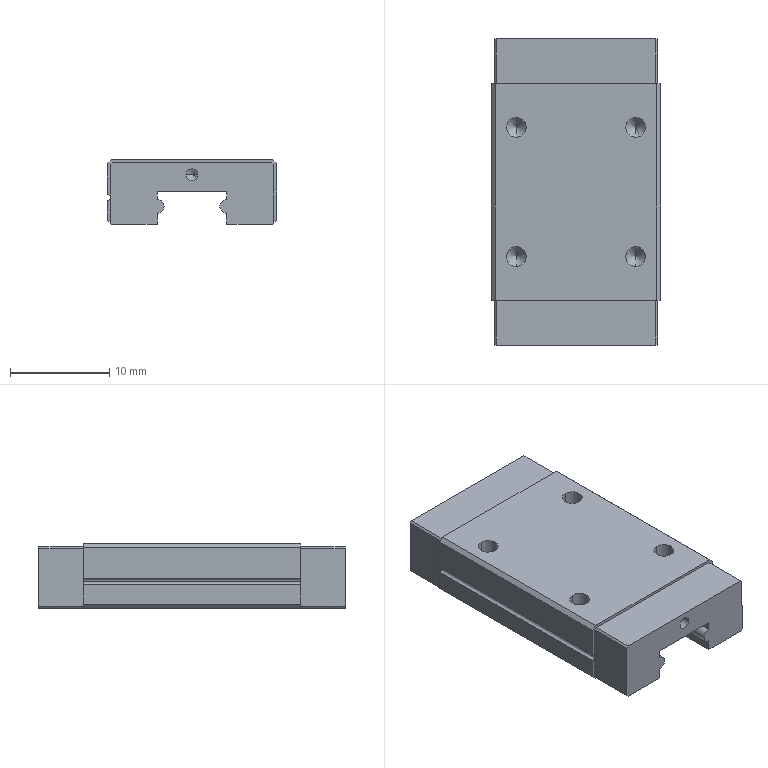Component | SolidWorks | MANIFOLD_SOLID_BREP_81-2 | 1 solid | 64 faces | volume 2602 mm3 | plane 35 | cylinder 17 | cone 12 | commonest cylinder face diameters 2 x8 1.2 x4 1.4 x3 0.6 x2